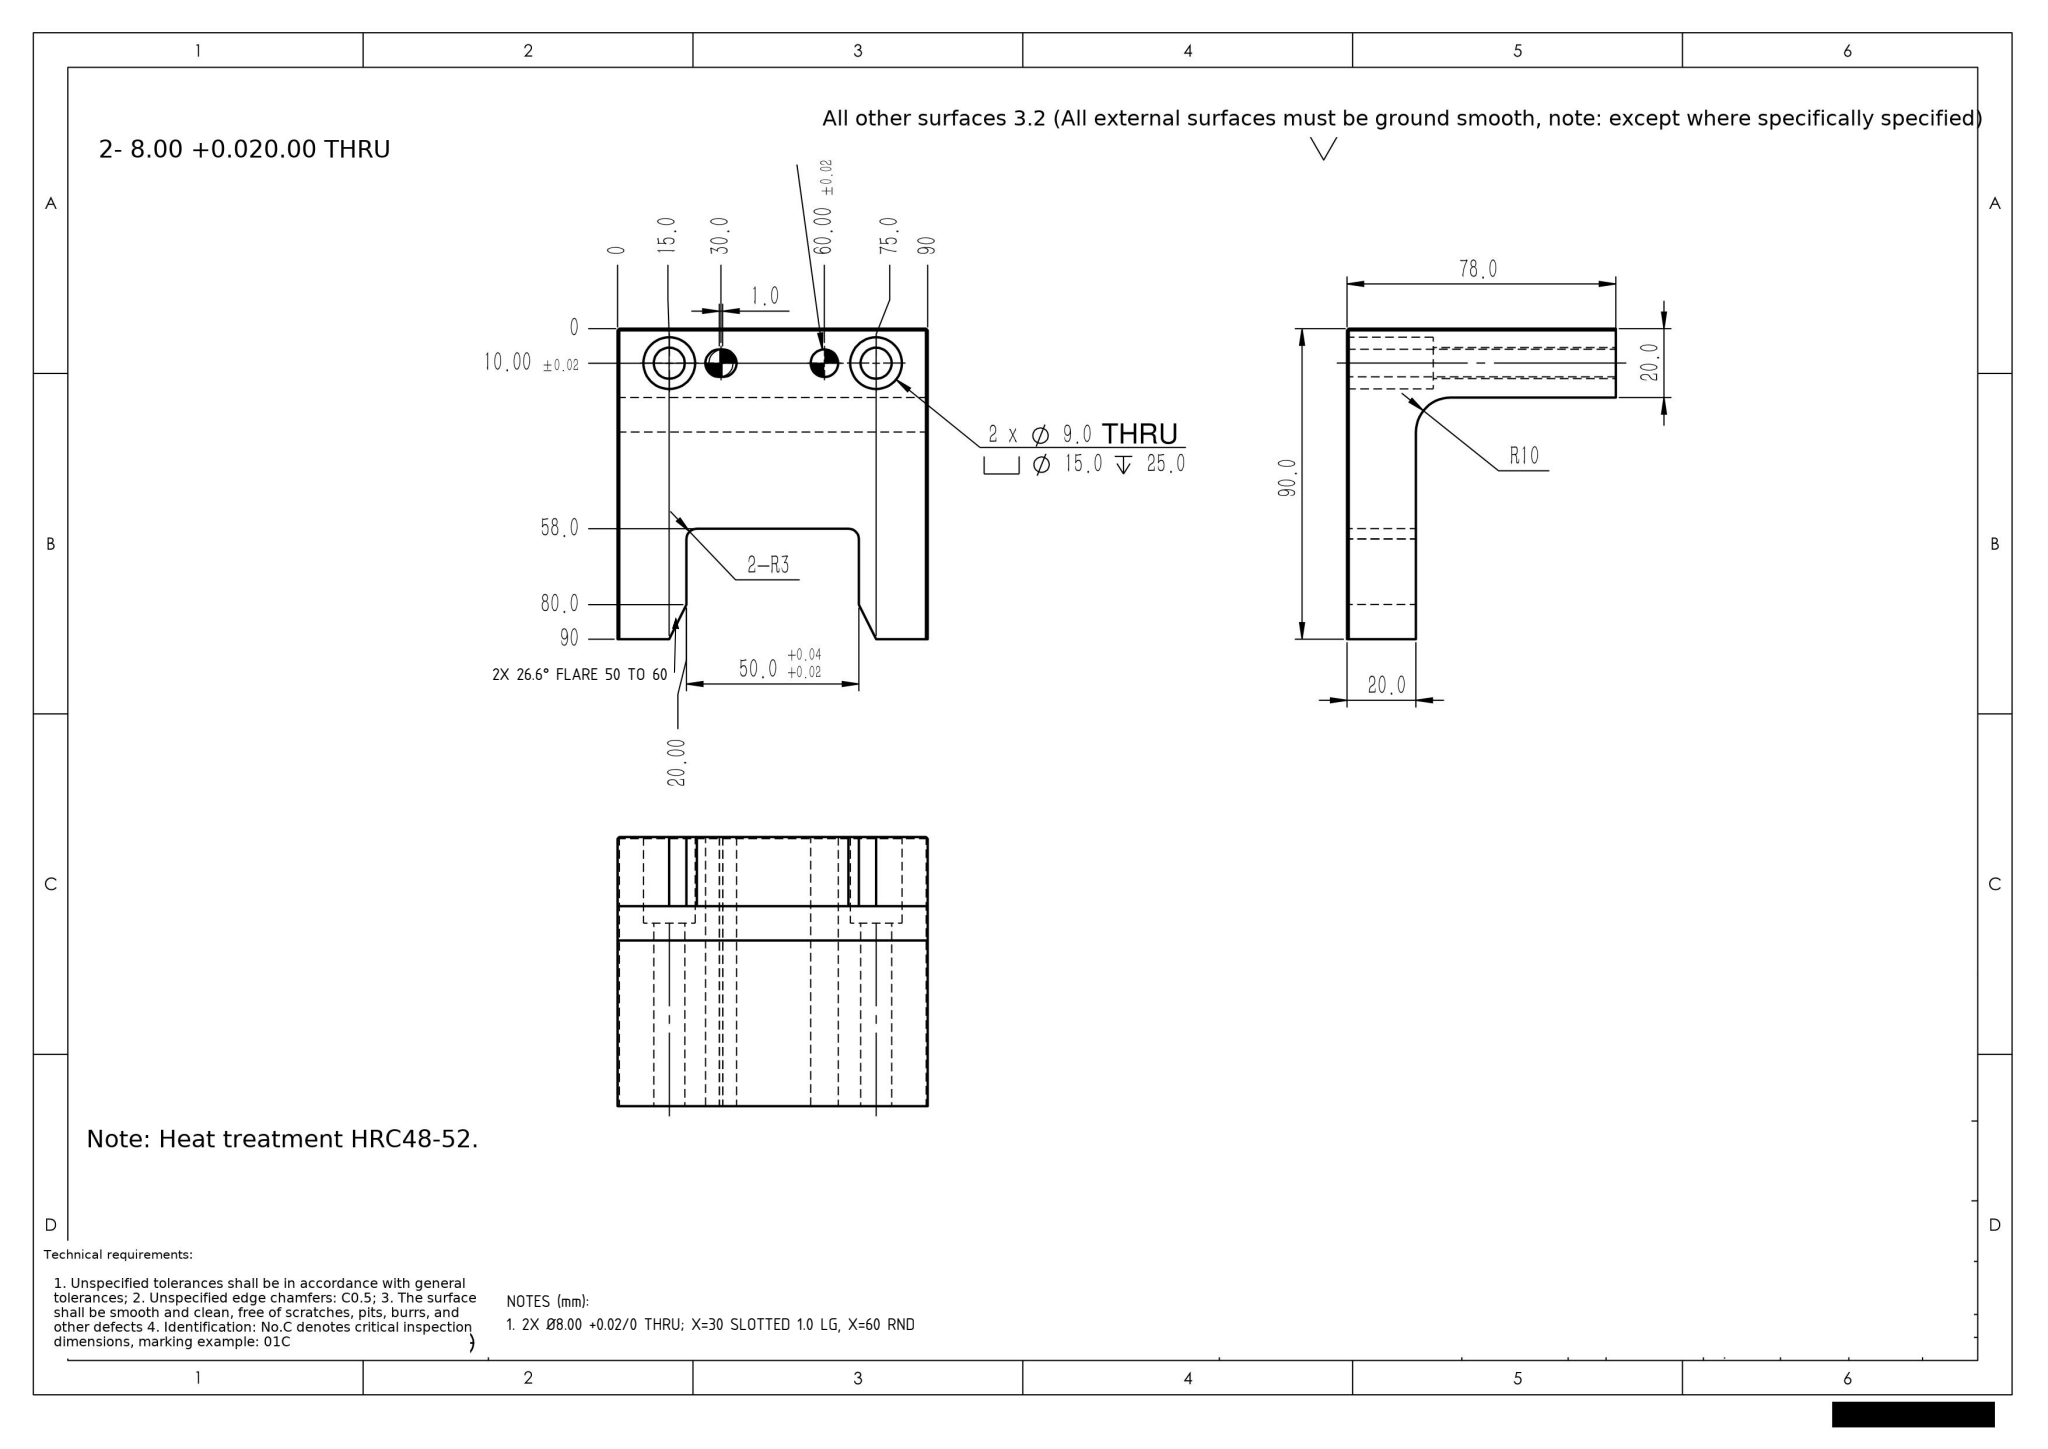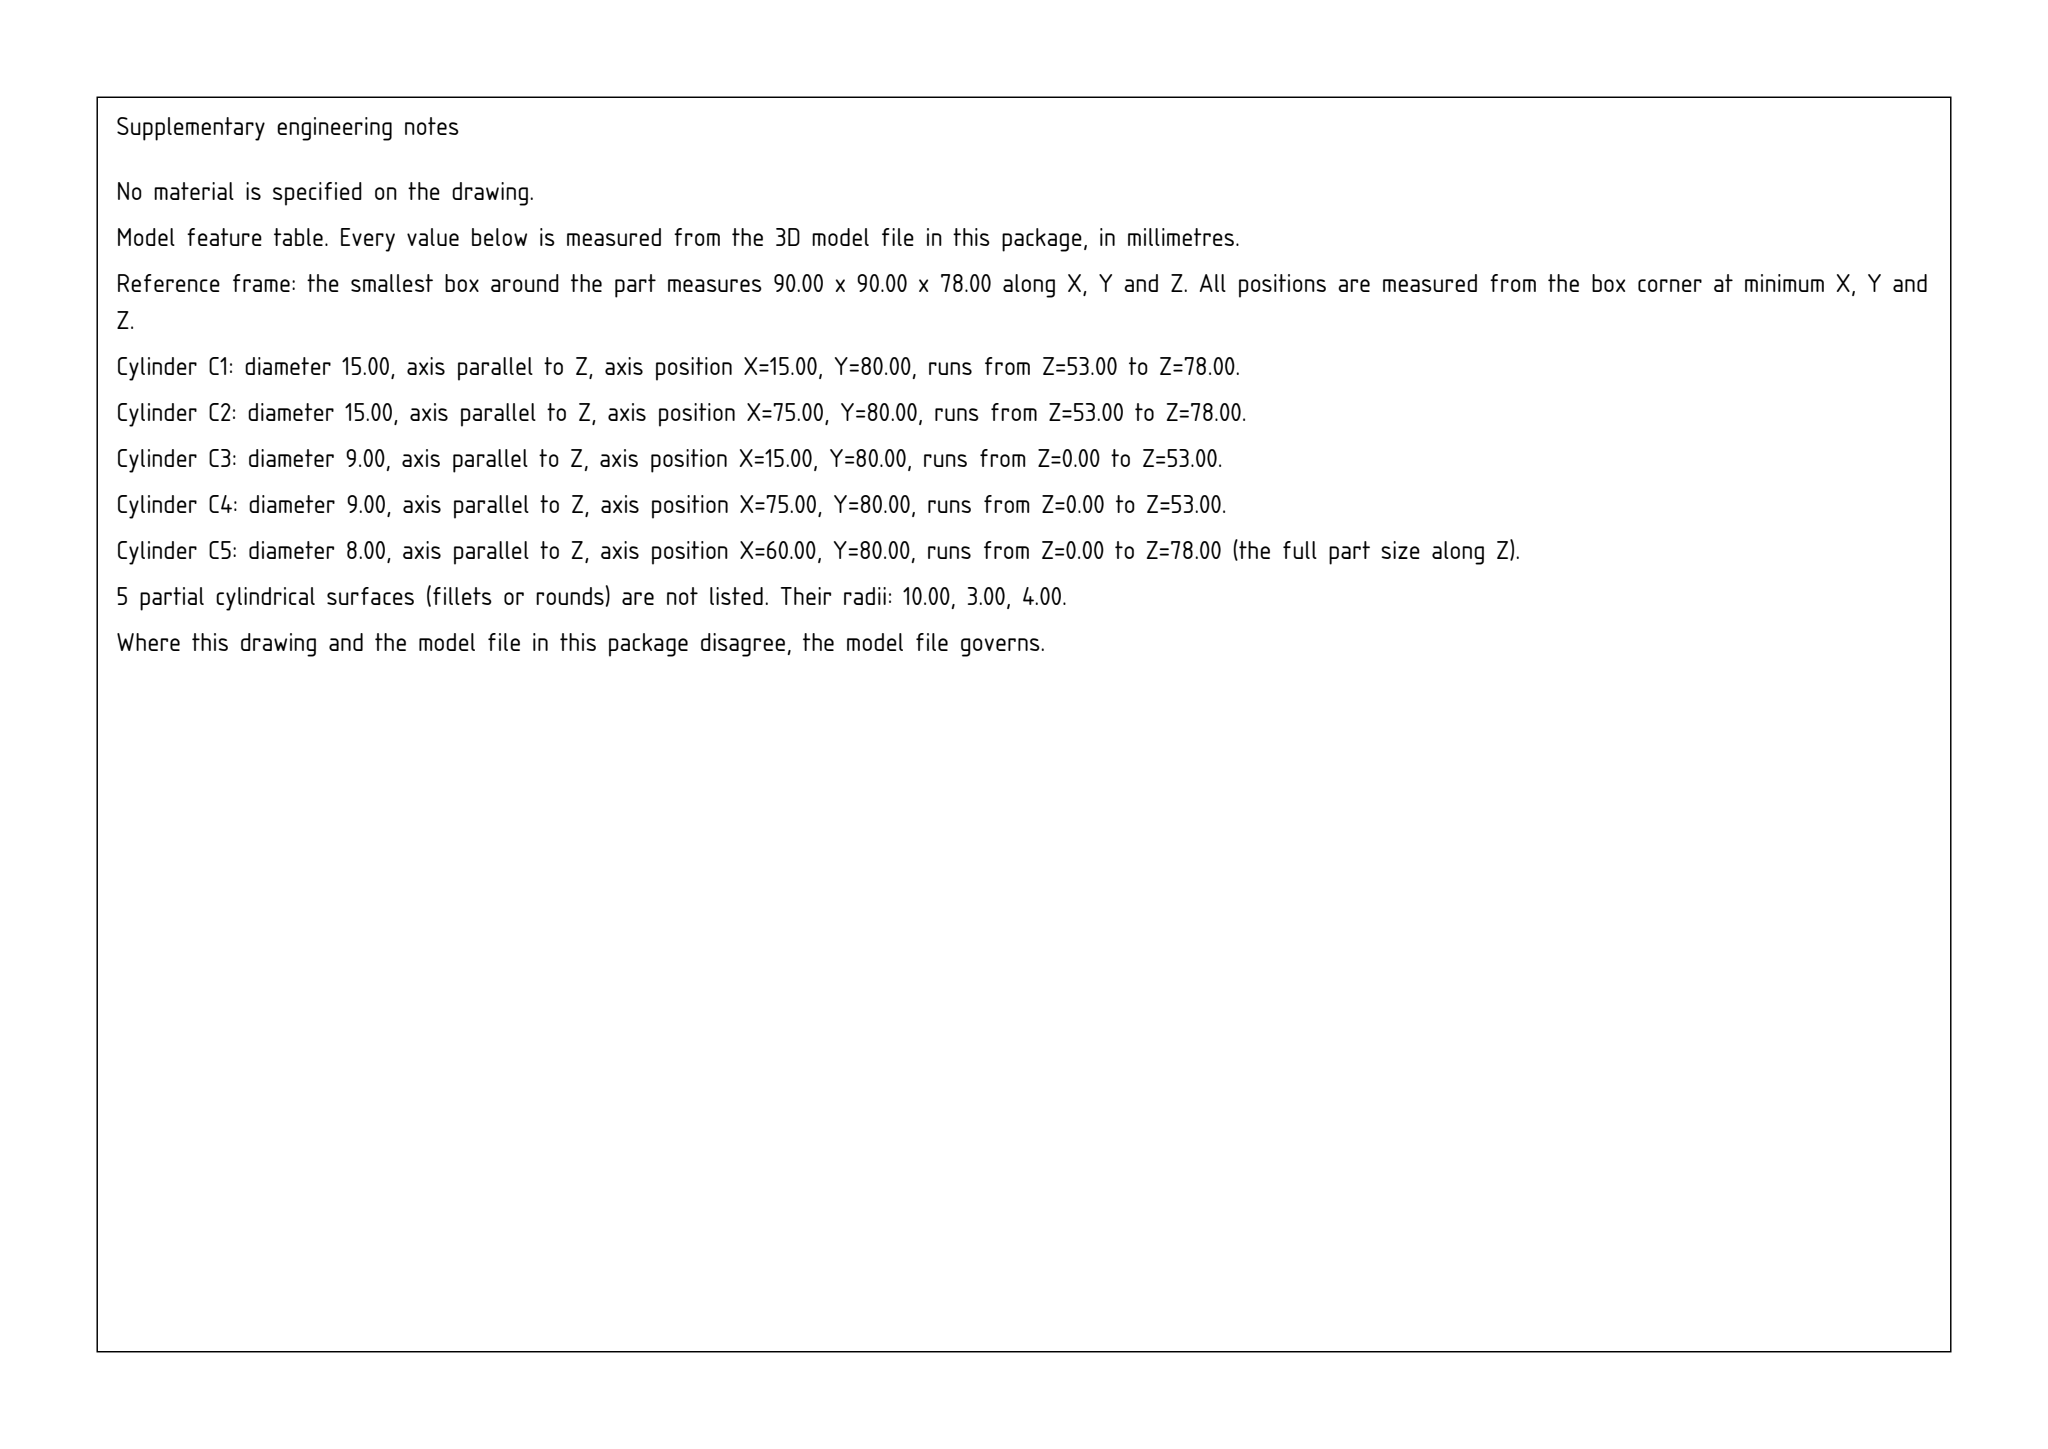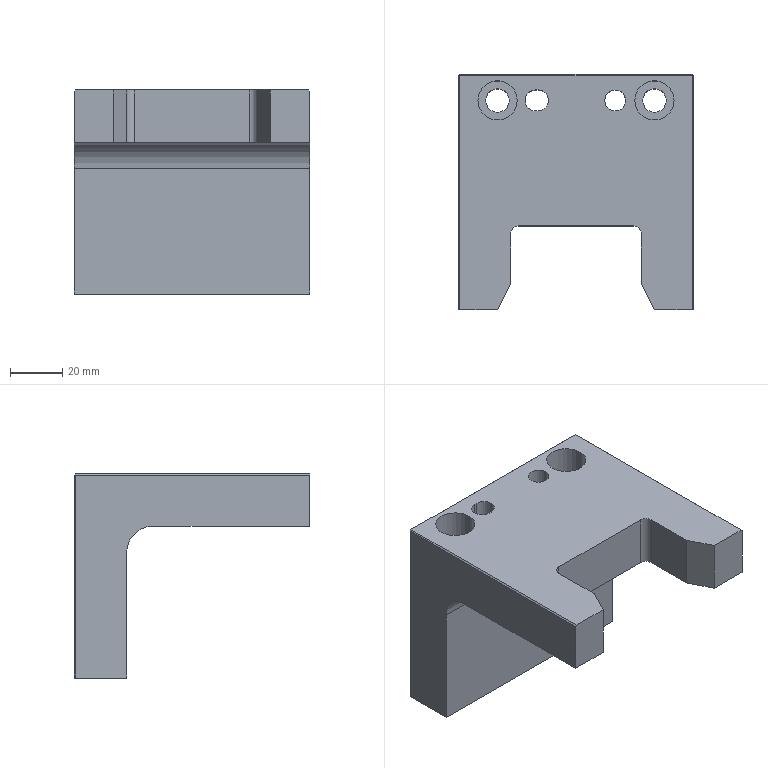Part | SolidWorks | mm | 1 solid | 41 faces | box 90 x 90 x 78 mm | volume 211311 mm3 | plane 25 | cylinder 16 | commonest cylinder face diameters 8 x5 15 x4 9 x4 6 x2 20 x1
Drawing notes:
2X Ø8.00 +0.02/0 THRU; X=30 SLOTTED 1.0 LG, X=60 RND | from the solid: hole/bore dia 8.0 axis z at [60.0,80.0] from 0.0 to 78.0 (THRU); two 180° dia 8.0 arcs at [29.5,80.0] and [30.5,80.0] from 0.0 to 78.0 form 1.0 long slot; y=80 is 10.00 from top edge
NOTCH MOUTH FLARE 2X 26.6 DEG: 50 OPENS TO 60 BTWN 80.0 AND 90 | from the solid: inclined_planes 26.6 deg, bbox_from [15,0,58] & [70,0,58], size [5,10,20]; notch walls x=20 & x=70 (50 wide) flare 5 each side to x=15/75 (60 wide) over y 0-10 i.e. drawing levels 80.0 to 90
build123d program:
from build123d import *

# Parameters (mm, degrees)
SKETCH1_W                                       = 90
SKETCH1_H                                       = 90
BOSS_EXTRUDE1_DEPTH                             = 10
F_9_0_9_DIAMETER_HOLE1_D                        = 9
SKETCH4_R                                       = 4
CUT_EXTRUDE1_DEPTH                              = 67.708
SKETCH5_W                                       = 50
SKETCH5_H                                       = 32
CUT_EXTRUDE2_DEPTH                              = 67.708
CUT_EXTRUDE3_DEPTH                              = 67.708
FILLET1_R                                       = 3
SKETCH7_W                                       = 90
SKETCH7_H                                       = 20
BOSS_EXTRUDE2_DEPTH                             = 58
M8_HEX_SOCKET_HEAD_CAP_SCREW_CBORE1_D           = 9
M8_HEX_SOCKET_HEAD_CAP_SCREW_CBORE1_CBORE_D     = 15
M8_HEX_SOCKET_HEAD_CAP_SCREW_CBORE1_CBORE_DEPTH = 25
CHAMFER1_SIZE                                   = 0.5
SKETCH11_R                                      = 4
CUT_EXTRUDE4_DEPTH                              = 87.105
FILLET2_R                                       = 10


with BuildPart() as part:
    # Sketch1 → Boss-Extrude1 (new, symmetric)
    with BuildSketch(Plane.XY):
        Rectangle(SKETCH1_W, SKETCH1_H)
    extrude(amount=BOSS_EXTRUDE1_DEPTH, both=True)

    # 9.0 _9_ Diameter Hole1 (through all)
    with Locations(Plane.XY.offset(10)):
        with Locations((30, 35), (-30, 35)):
            Hole(F_9_0_9_DIAMETER_HOLE1_D / 2)

    # Sketch4 → Cut-Extrude1 (cut, through all)
    with BuildSketch(Plane.XY.offset(10)):
        with Locations((15, 35)):
            Circle(SKETCH4_R)
        with BuildLine():
            Line((-14.5, 31), (-15.5, 31))
            ThreePointArc((-15.5, 31), (-19.5, 35), (-15.5, 39))
            Line((-15.5, 39), (-14.5, 39))
            ThreePointArc((-14.5, 39), (-10.5, 35), (-14.5, 31))
        make_face()
    extrude(amount=-CUT_EXTRUDE1_DEPTH, mode=Mode.SUBTRACT)

    # Sketch5 → Cut-Extrude2 (cut, through all)
    with BuildSketch(Plane.XY.offset(10)):
        with Locations((0, -29)):
            Rectangle(SKETCH5_W, SKETCH5_H)
    extrude(amount=-CUT_EXTRUDE2_DEPTH, mode=Mode.SUBTRACT)

    # Sketch6 → Cut-Extrude3 (cut, through all)
    with BuildSketch(Plane.XY.offset(10)):
        Polygon((25, -45), (25, -35), (30, -45), align=None)
        Polygon((-30, -45), (-25, -45), (-25, -35), align=None)
    extrude(amount=-CUT_EXTRUDE3_DEPTH, mode=Mode.SUBTRACT)

    # Fillet1
    fillet1_edges = [part.edges().sort_by_distance(p)[0] for p in [
        (-25, -13, 0),
        (25, -13, 0),
    ]]
    fillet(fillet1_edges, radius=FILLET1_R)

    # Sketch7 → Boss-Extrude2 (add)
    with BuildSketch(Plane(origin=(0, 0, -10), x_dir=(-1, 0, 0), z_dir=(0, 0, -1))):
        with Locations((0, 35)):
            Rectangle(SKETCH7_W, SKETCH7_H)
    extrude(amount=BOSS_EXTRUDE2_DEPTH)

    # M8 Hex Socket Head Cap Screw CBORE1 (through all)
    with Locations(Plane.XY.offset(10)):
        with Locations((-30, 35), (30, 35)):
            CounterBoreHole(M8_HEX_SOCKET_HEAD_CAP_SCREW_CBORE1_D / 2, M8_HEX_SOCKET_HEAD_CAP_SCREW_CBORE1_CBORE_D / 2, M8_HEX_SOCKET_HEAD_CAP_SCREW_CBORE1_CBORE_DEPTH)

    # Chamfer1
    chamfer1_edges = [part.edges().sort_by_distance(p)[0] for p in [
        (-45, 0, 10),
        (45, 0, 10),
        (0, 45, 10),
        (-45, 45, -29),
        (45, 45, -29),
    ]]
    chamfer(chamfer1_edges, length=CHAMFER1_SIZE)

    # Sketch11 → Cut-Extrude4 (cut, through all)
    with BuildSketch(Plane.XY.offset(-10)):
        with Locations((15, 35)):
            Circle(SKETCH11_R)
        with BuildLine():
            Line((-15.5, 31), (-14.5, 31))
            ThreePointArc((-14.5, 31), (-10.5, 35), (-14.5, 39))
            Line((-14.5, 39), (-15.5, 39))
            ThreePointArc((-15.5, 39), (-19.5, 35), (-15.5, 31))
        make_face()
    extrude(amount=-CUT_EXTRUDE4_DEPTH, mode=Mode.SUBTRACT)

    # Fillet2
    fillet2_edges = [part.edges().sort_by_distance(p)[0] for p in [
        (0, 25, -10),
    ]]
    fillet(fillet2_edges, radius=FILLET2_R)


solid = part.part